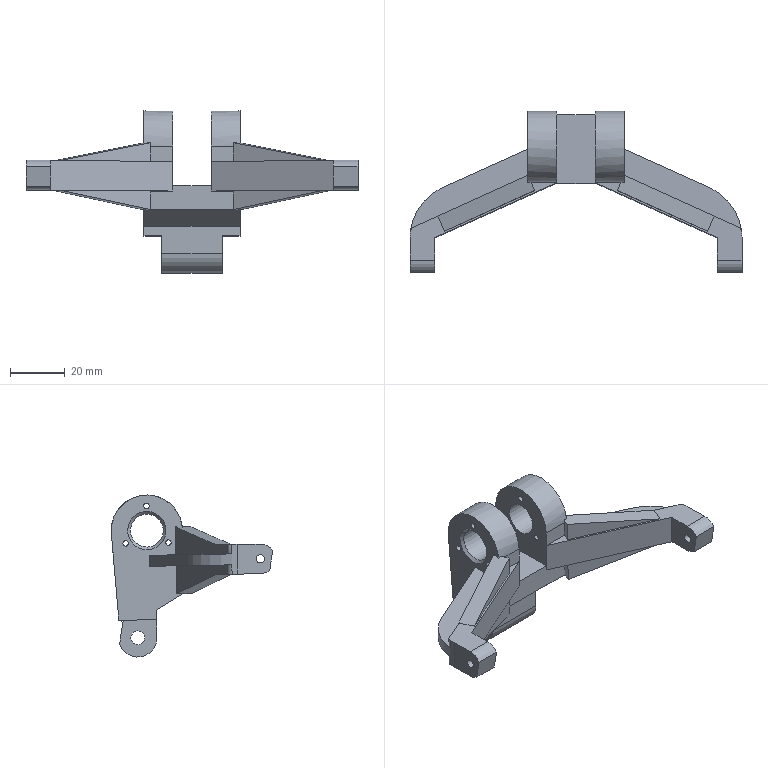Component | NX | ROTOR_BASE_ACC | 1 solid | 78 faces | volume 42003 mm3 | plane 52 | cylinder 24 | cone 2 | commonest cylinder face diameters 2 x6 10.8 x4 4 x4 3 x2 40 x2 26 x2 12 x2 14 x1